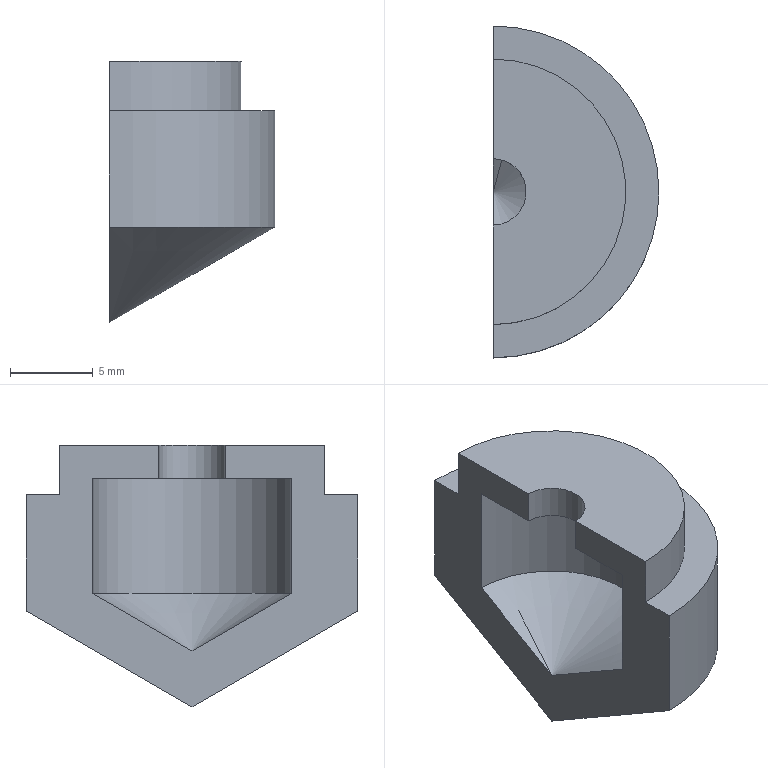Component | NX | VALVE_DISC | 1 solid | 10 faces | box 10 x 20 x 15.77 mm | volume 1233 mm3 | cylinder 4 | plane 4 | cone 2 | commonest cylinder face diameters 20 x1 12 x1 4 x1 16 x1
STEP:
#1=CARTESIAN_POINT('',(0.,0.,0.));
#2=DIRECTION('',(0.,0.,1.));
#3=DIRECTION('',(1.,0.,0.));
#4=AXIS2_PLACEMENT_3D('',#1,#2,#3);
#5=CARTESIAN_POINT('',(-146.777,10.,62.492));
#6=VERTEX_POINT('',#5);
#7=CARTESIAN_POINT('',(-146.777,-10.,62.492));
#8=VERTEX_POINT('',#7);
#9=CARTESIAN_POINT('',(-146.777,0.,62.492));
#10=DIRECTION('',(0.,0.,-1.));
#11=DIRECTION('',(0.,-1.,0.));
#12=AXIS2_PLACEMENT_3D('',#9,#10,#11);
#13=CIRCLE('',#12,10.);
#14=CARTESIAN_POINT('',(-146.777,0.,62.492));
#15=DIRECTION('',(0.,0.,-1.));
#16=DIRECTION('',(0.,-1.,0.));
#17=AXIS2_PLACEMENT_3D('',#14,#15,#16);
#18=CYLINDRICAL_SURFACE('',#17,10.);
#19=CARTESIAN_POINT('',(0.,0.));
#20=DIRECTION('',(1.,0.));
#21=VECTOR('',#20,1.);
#22=LINE('',#19,#21);
#23=(GEOMETRIC_REPRESENTATION_CONTEXT(2)PARAMETRIC_REPRESENTATION_CONTEXT()REPRESENTATION_CONTEXT('',''));
#24=DEFINITIONAL_REPRESENTATION('',(#22),#23);
#25=PCURVE('',#18,#24);
#26=CARTESIAN_POINT('',(-146.777,0.,62.492));
#27=DIRECTION('',(0.,0.,1.));
#28=DIRECTION('',(0.,1.,0.));
#29=AXIS2_PLACEMENT_3D('',#26,#27,#28);
#30=CONICAL_SURFACE('',#29,10.,1.047);
#31=CARTESIAN_POINT('',(9.425,0.));
#32=DIRECTION('',(-1.,0.));
#33=VECTOR('',#32,1.);
#34=LINE('',#31,#33);
#35=(GEOMETRIC_REPRESENTATION_CONTEXT(2)PARAMETRIC_REPRESENTATION_CONTEXT()REPRESENTATION_CONTEXT('',''));
#36=DEFINITIONAL_REPRESENTATION('',(#34),#35);
#37=PCURVE('',#30,#36);
#38=SURFACE_CURVE('',#13,(#25,#37),.PCURVE_S1.);
#39=EDGE_CURVE('',#6,#8,#38,.T.);
#40=ORIENTED_EDGE('',*,*,#39,.F.);
#41=CARTESIAN_POINT('',(-146.777,10.,69.492));
#42=VERTEX_POINT('',#41);
#43=CARTESIAN_POINT('',(-146.777,10.,69.492));
#44=DIRECTION('',(0.,0.,-1.));
#45=VECTOR('',#44,1.);
#46=LINE('',#43,#45);
#47=CARTESIAN_POINT('',(3.142,-7.));
#48=DIRECTION('',(0.,1.));
#49=VECTOR('',#48,1.);
#50=LINE('',#47,#49);
#51=(GEOMETRIC_REPRESENTATION_CONTEXT(2)PARAMETRIC_REPRESENTATION_CONTEXT()REPRESENTATION_CONTEXT('',''));
#52=DEFINITIONAL_REPRESENTATION('',(#50),#51);
#53=PCURVE('',#18,#52);
#54=CARTESIAN_POINT('',(-146.777,0.,62.492));
#55=DIRECTION('',(-1.,0.,0.));
#56=DIRECTION('',(-0.,-1.,0.));
#57=AXIS2_PLACEMENT_3D('',#54,#55,#56);
#58=PLANE('',#57);
#59=CARTESIAN_POINT('',(-10.,7.));
#60=DIRECTION('',(-0.,-1.));
#61=VECTOR('',#60,1.);
#62=LINE('',#59,#61);
#63=(GEOMETRIC_REPRESENTATION_CONTEXT(2)PARAMETRIC_REPRESENTATION_CONTEXT()REPRESENTATION_CONTEXT('',''));
#64=DEFINITIONAL_REPRESENTATION('',(#62),#63);
#65=PCURVE('',#58,#64);
#66=SURFACE_CURVE('',#46,(#53,#65),.PCURVE_S1.);
#67=EDGE_CURVE('',#42,#6,#66,.T.);
#68=ORIENTED_EDGE('',*,*,#67,.F.);
#69=CARTESIAN_POINT('',(-146.777,-10.,69.492));
#70=VERTEX_POINT('',#69);
#71=CARTESIAN_POINT('',(-146.777,0.,69.492));
#72=DIRECTION('',(0.,0.,-1.));
#73=DIRECTION('',(0.,-1.,0.));
#74=AXIS2_PLACEMENT_3D('',#71,#72,#73);
#75=CIRCLE('',#74,10.);
#76=CARTESIAN_POINT('',(0.,-7.));
#77=DIRECTION('',(1.,0.));
#78=VECTOR('',#77,1.);
#79=LINE('',#76,#78);
#80=(GEOMETRIC_REPRESENTATION_CONTEXT(2)PARAMETRIC_REPRESENTATION_CONTEXT()REPRESENTATION_CONTEXT('',''));
#81=DEFINITIONAL_REPRESENTATION('',(#79),#80);
#82=PCURVE('',#18,#81);
#83=CARTESIAN_POINT('',(-146.777,8.,69.492));
#84=DIRECTION('',(0.,0.,-1.));
#85=DIRECTION('',(0.,-1.,0.));
#86=AXIS2_PLACEMENT_3D('',#83,#84,#85);
#87=PLANE('',#86);
#88=CARTESIAN_POINT('',(8.,0.));
#89=DIRECTION('',(1.,0.));
#90=AXIS2_PLACEMENT_2D('',#88,#89);
#91=CIRCLE('',#90,10.);
#92=(GEOMETRIC_REPRESENTATION_CONTEXT(2)PARAMETRIC_REPRESENTATION_CONTEXT()REPRESENTATION_CONTEXT('',''));
#93=DEFINITIONAL_REPRESENTATION('',(#91),#92);
#94=PCURVE('',#87,#93);
#95=SURFACE_CURVE('',#75,(#82,#94),.PCURVE_S1.);
#96=EDGE_CURVE('',#42,#70,#95,.T.);
#97=ORIENTED_EDGE('',*,*,#96,.T.);
#98=CARTESIAN_POINT('',(-146.777,-10.,69.492));
#99=DIRECTION('',(-0.,0.,1.));
#100=VECTOR('',#99,1.);
#101=LINE('',#98,#100);
#102=CARTESIAN_POINT('',(6.283,-7.));
#103=DIRECTION('',(0.,-1.));
#104=VECTOR('',#103,1.);
#105=LINE('',#102,#104);
#106=(GEOMETRIC_REPRESENTATION_CONTEXT(2)PARAMETRIC_REPRESENTATION_CONTEXT()REPRESENTATION_CONTEXT('',''));
#107=DEFINITIONAL_REPRESENTATION('',(#105),#106);
#108=PCURVE('',#18,#107);
#109=CARTESIAN_POINT('',(10.,7.));
#110=DIRECTION('',(-0.,1.));
#111=VECTOR('',#110,1.);
#112=LINE('',#109,#111);
#113=(GEOMETRIC_REPRESENTATION_CONTEXT(2)PARAMETRIC_REPRESENTATION_CONTEXT()REPRESENTATION_CONTEXT('',''));
#114=DEFINITIONAL_REPRESENTATION('',(#112),#113);
#115=PCURVE('',#58,#114);
#116=SURFACE_CURVE('',#101,(#108,#115),.PCURVE_S1.);
#117=EDGE_CURVE('',#8,#70,#116,.T.);
#118=ORIENTED_EDGE('',*,*,#117,.F.);
#119=EDGE_LOOP('',(#40,#68,#97,#118));
#120=FACE_BOUND('',#119,.T.);
#121=ADVANCED_FACE('',(#120),#18,.T.);
#122=CARTESIAN_POINT('',(-146.777,0.,56.718));
#123=VERTEX_POINT('',#122);
#124=CARTESIAN_POINT('',(-146.777,-10.,62.492));
#125=DIRECTION('',(0.,-0.866,0.5));
#126=VECTOR('',#125,1.);
#127=LINE('',#124,#126);
#128=CARTESIAN_POINT('',(3.142,0.));
#129=DIRECTION('',(0.,1.));
#130=VECTOR('',#129,1.);
#131=LINE('',#128,#130);
#132=(GEOMETRIC_REPRESENTATION_CONTEXT(2)PARAMETRIC_REPRESENTATION_CONTEXT()REPRESENTATION_CONTEXT('',''));
#133=DEFINITIONAL_REPRESENTATION('',(#131),#132);
#134=PCURVE('',#30,#133);
#135=CARTESIAN_POINT('',(10.,0.));
#136=DIRECTION('',(0.866,0.5));
#137=VECTOR('',#136,1.);
#138=LINE('',#135,#137);
#139=(GEOMETRIC_REPRESENTATION_CONTEXT(2)PARAMETRIC_REPRESENTATION_CONTEXT()REPRESENTATION_CONTEXT('',''));
#140=DEFINITIONAL_REPRESENTATION('',(#138),#139);
#141=PCURVE('',#58,#140);
#142=SURFACE_CURVE('',#127,(#134,#141),.PCURVE_S1.);
#143=EDGE_CURVE('',#123,#8,#142,.T.);
#144=ORIENTED_EDGE('',*,*,#143,.F.);
#145=CARTESIAN_POINT('',(-146.777,10.,62.492));
#146=DIRECTION('',(-0.,-0.866,-0.5));
#147=VECTOR('',#146,1.);
#148=LINE('',#145,#147);
#149=CARTESIAN_POINT('',(6.283,0.));
#150=DIRECTION('',(0.,-1.));
#151=VECTOR('',#150,1.);
#152=LINE('',#149,#151);
#153=(GEOMETRIC_REPRESENTATION_CONTEXT(2)PARAMETRIC_REPRESENTATION_CONTEXT()REPRESENTATION_CONTEXT('',''));
#154=DEFINITIONAL_REPRESENTATION('',(#152),#153);
#155=PCURVE('',#30,#154);
#156=CARTESIAN_POINT('',(-10.,0.));
#157=DIRECTION('',(0.866,-0.5));
#158=VECTOR('',#157,1.);
#159=LINE('',#156,#158);
#160=(GEOMETRIC_REPRESENTATION_CONTEXT(2)PARAMETRIC_REPRESENTATION_CONTEXT()REPRESENTATION_CONTEXT('',''));
#161=DEFINITIONAL_REPRESENTATION('',(#159),#160);
#162=PCURVE('',#58,#161);
#163=SURFACE_CURVE('',#148,(#155,#162),.PCURVE_S1.);
#164=EDGE_CURVE('',#6,#123,#163,.T.);
#165=ORIENTED_EDGE('',*,*,#164,.F.);
#166=ORIENTED_EDGE('',*,*,#39,.T.);
#167=EDGE_LOOP('',(#144,#165,#166));
#168=FACE_BOUND('',#167,.T.);
#169=ADVANCED_FACE('',(#168),#30,.T.);
#170=CARTESIAN_POINT('',(-146.777,-6.,63.557));
#171=VERTEX_POINT('',#170);
#172=CARTESIAN_POINT('',(-146.777,0.,60.093));
#173=VERTEX_POINT('',#172);
#174=CARTESIAN_POINT('',(-146.777,0.,60.093));
#175=DIRECTION('',(-0.,0.866,-0.5));
#176=VECTOR('',#175,1.);
#177=LINE('',#174,#176);
#178=CARTESIAN_POINT('',(-146.777,0.,60.093));
#179=DIRECTION('',(0.,0.,1.));
#180=DIRECTION('',(0.,1.,0.));
#181=AXIS2_PLACEMENT_3D('',#178,#179,#180);
#182=CONICAL_SURFACE('',#181,0.,1.047);
#183=CARTESIAN_POINT('',(3.142,0.));
#184=DIRECTION('',(0.,-1.));
#185=VECTOR('',#184,1.);
#186=LINE('',#183,#185);
#187=(GEOMETRIC_REPRESENTATION_CONTEXT(2)PARAMETRIC_REPRESENTATION_CONTEXT()REPRESENTATION_CONTEXT('',''));
#188=DEFINITIONAL_REPRESENTATION('',(#186),#187);
#189=PCURVE('',#182,#188);
#190=CARTESIAN_POINT('',(0.,-2.398));
#191=DIRECTION('',(-0.866,-0.5));
#192=VECTOR('',#191,1.);
#193=LINE('',#190,#192);
#194=(GEOMETRIC_REPRESENTATION_CONTEXT(2)PARAMETRIC_REPRESENTATION_CONTEXT()REPRESENTATION_CONTEXT('',''));
#195=DEFINITIONAL_REPRESENTATION('',(#193),#194);
#196=PCURVE('',#58,#195);
#197=SURFACE_CURVE('',#177,(#189,#196),.PCURVE_S1.);
#198=EDGE_CURVE('',#171,#173,#197,.T.);
#199=ORIENTED_EDGE('',*,*,#198,.T.);
#200=CARTESIAN_POINT('',(-146.777,6.,63.557));
#201=VERTEX_POINT('',#200);
#202=CARTESIAN_POINT('',(-146.777,0.,60.093));
#203=DIRECTION('',(0.,0.866,0.5));
#204=VECTOR('',#203,1.);
#205=LINE('',#202,#204);
#206=CARTESIAN_POINT('',(6.283,-0.));
#207=CARTESIAN_POINT('',(6.283,0.05249));
#208=CARTESIAN_POINT('',(6.283,0.1575));
#209=CARTESIAN_POINT('',(6.283,0.3149));
#210=CARTESIAN_POINT('',(6.283,0.4724));
#211=CARTESIAN_POINT('',(6.283,0.6298));
#212=CARTESIAN_POINT('',(6.283,0.7873));
#213=CARTESIAN_POINT('',(6.283,0.9448));
#214=CARTESIAN_POINT('',(6.283,1.102));
#215=CARTESIAN_POINT('',(6.283,1.26));
#216=CARTESIAN_POINT('',(6.283,1.417));
#217=CARTESIAN_POINT('',(6.283,1.575));
#218=CARTESIAN_POINT('',(6.283,1.732));
#219=CARTESIAN_POINT('',(6.283,1.89));
#220=CARTESIAN_POINT('',(6.283,2.047));
#221=CARTESIAN_POINT('',(6.283,2.204));
#222=CARTESIAN_POINT('',(6.283,2.362));
#223=CARTESIAN_POINT('',(6.283,2.519));
#224=CARTESIAN_POINT('',(6.283,2.677));
#225=CARTESIAN_POINT('',(6.283,2.834));
#226=CARTESIAN_POINT('',(6.283,2.992));
#227=CARTESIAN_POINT('',(6.283,3.149));
#228=CARTESIAN_POINT('',(6.283,3.307));
#229=CARTESIAN_POINT('',(6.283,3.412));
#230=CARTESIAN_POINT('',(6.283,3.464));
#231=B_SPLINE_CURVE_WITH_KNOTS('',3,(#206,#207,#208,#209,#210,#211,#212,#213,#214,#215,#216,#217,#218,#219,#220,#221,#222,#223,#224,#225,#226,#227,#228,#229,#230),.UNSPECIFIED.,.F.,.F.,(4,1,1,1,1,1,1,1,1,1,1,1,1,1,1,1,1,1,1,1,1,1,4),(-0.,0.3149,0.6298,0.9448,1.26,1.575,1.89,2.204,2.519,2.834,3.149,3.464,3.779,4.094,4.409,4.724,5.039,5.354,5.669,5.983,6.298,6.613,6.928),.UNSPECIFIED.);
#232=(GEOMETRIC_REPRESENTATION_CONTEXT(2)PARAMETRIC_REPRESENTATION_CONTEXT()REPRESENTATION_CONTEXT('',''));
#233=DEFINITIONAL_REPRESENTATION('',(#231),#232);
#234=PCURVE('',#182,#233);
#235=CARTESIAN_POINT('',(0.,-2.398));
#236=DIRECTION('',(-0.866,0.5));
#237=VECTOR('',#236,1.);
#238=LINE('',#235,#237);
#239=(GEOMETRIC_REPRESENTATION_CONTEXT(2)PARAMETRIC_REPRESENTATION_CONTEXT()REPRESENTATION_CONTEXT('',''));
#240=DEFINITIONAL_REPRESENTATION('',(#238),#239);
#241=PCURVE('',#58,#240);
#242=SURFACE_CURVE('',#205,(#234,#241),.PCURVE_S1.);
#243=EDGE_CURVE('',#173,#201,#242,.T.);
#244=ORIENTED_EDGE('',*,*,#243,.T.);
#245=CARTESIAN_POINT('',(-146.777,0.,63.557));
#246=DIRECTION('',(0.,0.,-1.));
#247=DIRECTION('',(0.,-1.,0.));
#248=AXIS2_PLACEMENT_3D('',#245,#246,#247);
#249=CIRCLE('',#248,6.);
#250=CARTESIAN_POINT('',(9.425,3.464));
#251=DIRECTION('',(-1.,0.));
#252=VECTOR('',#251,1.);
#253=LINE('',#250,#252);
#254=(GEOMETRIC_REPRESENTATION_CONTEXT(2)PARAMETRIC_REPRESENTATION_CONTEXT()REPRESENTATION_CONTEXT('',''));
#255=DEFINITIONAL_REPRESENTATION('',(#253),#254);
#256=PCURVE('',#182,#255);
#257=CARTESIAN_POINT('',(-146.777,0.,62.492));
#258=DIRECTION('',(0.,0.,-1.));
#259=DIRECTION('',(0.,-1.,0.));
#260=AXIS2_PLACEMENT_3D('',#257,#258,#259);
#261=CYLINDRICAL_SURFACE('',#260,6.);
#262=CARTESIAN_POINT('',(0.,-1.066));
#263=DIRECTION('',(1.,0.));
#264=VECTOR('',#263,1.);
#265=LINE('',#262,#264);
#266=(GEOMETRIC_REPRESENTATION_CONTEXT(2)PARAMETRIC_REPRESENTATION_CONTEXT()REPRESENTATION_CONTEXT('',''));
#267=DEFINITIONAL_REPRESENTATION('',(#265),#266);
#268=PCURVE('',#261,#267);
#269=SURFACE_CURVE('',#249,(#256,#268),.PCURVE_S1.);
#270=EDGE_CURVE('',#201,#171,#269,.T.);
#271=ORIENTED_EDGE('',*,*,#270,.T.);
#272=EDGE_LOOP('',(#199,#244,#271));
#273=FACE_BOUND('',#272,.F.);
#274=ADVANCED_FACE('',(#273),#182,.F.);
#275=CARTESIAN_POINT('',(-146.777,-6.,70.492));
#276=VERTEX_POINT('',#275);
#277=CARTESIAN_POINT('',(-146.777,-6.,63.557));
#278=DIRECTION('',(-0.,0.,-1.));
#279=VECTOR('',#278,1.);
#280=LINE('',#277,#279);
#281=CARTESIAN_POINT('',(6.283,-1.066));
#282=DIRECTION('',(0.,1.));
#283=VECTOR('',#282,1.);
#284=LINE('',#281,#283);
#285=(GEOMETRIC_REPRESENTATION_CONTEXT(2)PARAMETRIC_REPRESENTATION_CONTEXT()REPRESENTATION_CONTEXT('',''));
#286=DEFINITIONAL_REPRESENTATION('',(#284),#285);
#287=PCURVE('',#261,#286);
#288=CARTESIAN_POINT('',(6.,1.066));
#289=DIRECTION('',(-0.,-1.));
#290=VECTOR('',#289,1.);
#291=LINE('',#288,#290);
#292=(GEOMETRIC_REPRESENTATION_CONTEXT(2)PARAMETRIC_REPRESENTATION_CONTEXT()REPRESENTATION_CONTEXT('',''));
#293=DEFINITIONAL_REPRESENTATION('',(#291),#292);
#294=PCURVE('',#58,#293);
#295=SURFACE_CURVE('',#280,(#287,#294),.PCURVE_S1.);
#296=EDGE_CURVE('',#276,#171,#295,.T.);
#297=ORIENTED_EDGE('',*,*,#296,.T.);
#298=ORIENTED_EDGE('',*,*,#270,.F.);
#299=CARTESIAN_POINT('',(-146.777,6.,70.492));
#300=VERTEX_POINT('',#299);
#301=CARTESIAN_POINT('',(-146.777,6.,63.557));
#302=DIRECTION('',(0.,0.,1.));
#303=VECTOR('',#302,1.);
#304=LINE('',#301,#303);
#305=CARTESIAN_POINT('',(3.142,-1.066));
#306=DIRECTION('',(0.,-1.));
#307=VECTOR('',#306,1.);
#308=LINE('',#305,#307);
#309=(GEOMETRIC_REPRESENTATION_CONTEXT(2)PARAMETRIC_REPRESENTATION_CONTEXT()REPRESENTATION_CONTEXT('',''));
#310=DEFINITIONAL_REPRESENTATION('',(#308),#309);
#311=PCURVE('',#261,#310);
#312=CARTESIAN_POINT('',(-6.,1.066));
#313=DIRECTION('',(-0.,1.));
#314=VECTOR('',#313,1.);
#315=LINE('',#312,#314);
#316=(GEOMETRIC_REPRESENTATION_CONTEXT(2)PARAMETRIC_REPRESENTATION_CONTEXT()REPRESENTATION_CONTEXT('',''));
#317=DEFINITIONAL_REPRESENTATION('',(#315),#316);
#318=PCURVE('',#58,#317);
#319=SURFACE_CURVE('',#304,(#311,#318),.PCURVE_S1.);
#320=EDGE_CURVE('',#201,#300,#319,.T.);
#321=ORIENTED_EDGE('',*,*,#320,.T.);
#322=CARTESIAN_POINT('',(-146.777,0.,70.492));
#323=DIRECTION('',(0.,0.,-1.));
#324=DIRECTION('',(0.,-1.,0.));
#325=AXIS2_PLACEMENT_3D('',#322,#323,#324);
#326=CIRCLE('',#325,6.);
#327=CARTESIAN_POINT('',(0.,-8.));
#328=DIRECTION('',(1.,0.));
#329=VECTOR('',#328,1.);
#330=LINE('',#327,#329);
#331=(GEOMETRIC_REPRESENTATION_CONTEXT(2)PARAMETRIC_REPRESENTATION_CONTEXT()REPRESENTATION_CONTEXT('',''));
#332=DEFINITIONAL_REPRESENTATION('',(#330),#331);
#333=PCURVE('',#261,#332);
#334=CARTESIAN_POINT('',(-146.777,6.,70.492));
#335=DIRECTION('',(0.,0.,1.));
#336=DIRECTION('',(0.,1.,0.));
#337=AXIS2_PLACEMENT_3D('',#334,#335,#336);
#338=PLANE('',#337);
#339=CARTESIAN_POINT('',(-12.,0.));
#340=CARTESIAN_POINT('',(-12.,10.392));
#341=CARTESIAN_POINT('',(-3.,5.196));
#342=CARTESIAN_POINT('',(6.,0.));
#343=CARTESIAN_POINT('',(-3.,-5.196));
#344=CARTESIAN_POINT('',(-12.,-10.392));
#345=CARTESIAN_POINT('',(-12.,0.));
#346=(BOUNDED_CURVE()B_SPLINE_CURVE(2,(#339,#340,#341,#342,#343,#344,#345),.UNSPECIFIED.,.T.,.F.)B_SPLINE_CURVE_WITH_KNOTS((1,2,2,2,2,1),(-2.094,0.,2.094,4.189,6.283,8.378),.UNSPECIFIED.)CURVE()GEOMETRIC_REPRESENTATION_ITEM()RATIONAL_B_SPLINE_CURVE((1.,0.5,1.,0.5,1.,0.5,1.))REPRESENTATION_ITEM(''));
#347=(GEOMETRIC_REPRESENTATION_CONTEXT(2)PARAMETRIC_REPRESENTATION_CONTEXT()REPRESENTATION_CONTEXT('',''));
#348=DEFINITIONAL_REPRESENTATION('',(#346),#347);
#349=PCURVE('',#338,#348);
#350=SURFACE_CURVE('',#326,(#333,#349),.PCURVE_S1.);
#351=EDGE_CURVE('',#300,#276,#350,.T.);
#352=ORIENTED_EDGE('',*,*,#351,.T.);
#353=EDGE_LOOP('',(#297,#298,#321,#352));
#354=FACE_BOUND('',#353,.F.);
#355=ADVANCED_FACE('',(#354),#261,.F.);
#356=CARTESIAN_POINT('',(-146.777,2.,70.492));
#357=VERTEX_POINT('',#356);
#358=CARTESIAN_POINT('',(-146.777,-2.,70.492));
#359=VERTEX_POINT('',#358);
#360=CARTESIAN_POINT('',(-146.777,0.,70.492));
#361=DIRECTION('',(0.,0.,-1.));
#362=DIRECTION('',(0.,-1.,0.));
#363=AXIS2_PLACEMENT_3D('',#360,#361,#362);
#364=CIRCLE('',#363,2.);
#365=CARTESIAN_POINT('',(-8.,0.));
#366=CARTESIAN_POINT('',(-8.,3.464));
#367=CARTESIAN_POINT('',(-5.,1.732));
#368=CARTESIAN_POINT('',(-2.,0.));
#369=CARTESIAN_POINT('',(-5.,-1.732));
#370=CARTESIAN_POINT('',(-8.,-3.464));
#371=CARTESIAN_POINT('',(-8.,0.));
#372=(BOUNDED_CURVE()B_SPLINE_CURVE(2,(#365,#366,#367,#368,#369,#370,#371),.UNSPECIFIED.,.T.,.F.)B_SPLINE_CURVE_WITH_KNOTS((1,2,2,2,2,1),(-2.094,0.,2.094,4.189,6.283,8.378),.UNSPECIFIED.)CURVE()GEOMETRIC_REPRESENTATION_ITEM()RATIONAL_B_SPLINE_CURVE((1.,0.5,1.,0.5,1.,0.5,1.))REPRESENTATION_ITEM(''));
#373=(GEOMETRIC_REPRESENTATION_CONTEXT(2)PARAMETRIC_REPRESENTATION_CONTEXT()REPRESENTATION_CONTEXT('',''));
#374=DEFINITIONAL_REPRESENTATION('',(#372),#373);
#375=PCURVE('',#338,#374);
#376=CARTESIAN_POINT('',(-146.777,0.,62.492));
#377=DIRECTION('',(0.,0.,-1.));
#378=DIRECTION('',(0.,-1.,0.));
#379=AXIS2_PLACEMENT_3D('',#376,#377,#378);
#380=CYLINDRICAL_SURFACE('',#379,2.);
#381=CARTESIAN_POINT('',(0.,-8.));
#382=DIRECTION('',(1.,0.));
#383=VECTOR('',#382,1.);
#384=LINE('',#381,#383);
#385=(GEOMETRIC_REPRESENTATION_CONTEXT(2)PARAMETRIC_REPRESENTATION_CONTEXT()REPRESENTATION_CONTEXT('',''));
#386=DEFINITIONAL_REPRESENTATION('',(#384),#385);
#387=PCURVE('',#380,#386);
#388=SURFACE_CURVE('',#364,(#375,#387),.PCURVE_S1.);
#389=EDGE_CURVE('',#357,#359,#388,.T.);
#390=ORIENTED_EDGE('',*,*,#389,.F.);
#391=CARTESIAN_POINT('',(-146.777,6.,70.492));
#392=DIRECTION('',(-0.,-1.,-0.));
#393=VECTOR('',#392,1.);
#394=LINE('',#391,#393);
#395=CARTESIAN_POINT('',(0.,0.));
#396=DIRECTION('',(-1.,0.));
#397=VECTOR('',#396,1.);
#398=LINE('',#395,#397);
#399=(GEOMETRIC_REPRESENTATION_CONTEXT(2)PARAMETRIC_REPRESENTATION_CONTEXT()REPRESENTATION_CONTEXT('',''));
#400=DEFINITIONAL_REPRESENTATION('',(#398),#399);
#401=PCURVE('',#338,#400);
#402=CARTESIAN_POINT('',(-6.,8.));
#403=DIRECTION('',(1.,-0.));
#404=VECTOR('',#403,1.);
#405=LINE('',#402,#404);
#406=(GEOMETRIC_REPRESENTATION_CONTEXT(2)PARAMETRIC_REPRESENTATION_CONTEXT()REPRESENTATION_CONTEXT('',''));
#407=DEFINITIONAL_REPRESENTATION('',(#405),#406);
#408=PCURVE('',#58,#407);
#409=SURFACE_CURVE('',#394,(#401,#408),.PCURVE_S1.);
#410=EDGE_CURVE('',#300,#357,#409,.T.);
#411=ORIENTED_EDGE('',*,*,#410,.F.);
#412=ORIENTED_EDGE('',*,*,#351,.T.);
#413=CARTESIAN_POINT('',(-146.777,-6.,70.492));
#414=DIRECTION('',(0.,-1.,0.));
#415=VECTOR('',#414,1.);
#416=LINE('',#413,#415);
#417=CARTESIAN_POINT('',(-12.,0.));
#418=DIRECTION('',(-1.,-0.));
#419=VECTOR('',#418,1.);
#420=LINE('',#417,#419);
#421=(GEOMETRIC_REPRESENTATION_CONTEXT(2)PARAMETRIC_REPRESENTATION_CONTEXT()REPRESENTATION_CONTEXT('',''));
#422=DEFINITIONAL_REPRESENTATION('',(#420),#421);
#423=PCURVE('',#338,#422);
#424=CARTESIAN_POINT('',(6.,8.));
#425=DIRECTION('',(1.,0.));
#426=VECTOR('',#425,1.);
#427=LINE('',#424,#426);
#428=(GEOMETRIC_REPRESENTATION_CONTEXT(2)PARAMETRIC_REPRESENTATION_CONTEXT()REPRESENTATION_CONTEXT('',''));
#429=DEFINITIONAL_REPRESENTATION('',(#427),#428);
#430=PCURVE('',#58,#429);
#431=SURFACE_CURVE('',#416,(#423,#430),.PCURVE_S1.);
#432=EDGE_CURVE('',#359,#276,#431,.T.);
#433=ORIENTED_EDGE('',*,*,#432,.F.);
#434=EDGE_LOOP('',(#390,#411,#412,#433));
#435=FACE_BOUND('',#434,.T.);
#436=ADVANCED_FACE('',(#435),#338,.F.);
#437=CARTESIAN_POINT('',(-146.777,-2.,72.492));
#438=VERTEX_POINT('',#437);
#439=CARTESIAN_POINT('',(-146.777,-2.,70.492));
#440=DIRECTION('',(0.,-0.,-1.));
#441=VECTOR('',#440,1.);
#442=LINE('',#439,#441);
#443=CARTESIAN_POINT('',(6.283,-8.));
#444=DIRECTION('',(0.,1.));
#445=VECTOR('',#444,1.);
#446=LINE('',#443,#445);
#447=(GEOMETRIC_REPRESENTATION_CONTEXT(2)PARAMETRIC_REPRESENTATION_CONTEXT()REPRESENTATION_CONTEXT('',''));
#448=DEFINITIONAL_REPRESENTATION('',(#446),#447);
#449=PCURVE('',#380,#448);
#450=CARTESIAN_POINT('',(2.,8.));
#451=DIRECTION('',(0.,-1.));
#452=VECTOR('',#451,1.);
#453=LINE('',#450,#452);
#454=(GEOMETRIC_REPRESENTATION_CONTEXT(2)PARAMETRIC_REPRESENTATION_CONTEXT()REPRESENTATION_CONTEXT('',''));
#455=DEFINITIONAL_REPRESENTATION('',(#453),#454);
#456=PCURVE('',#58,#455);
#457=SURFACE_CURVE('',#442,(#449,#456),.PCURVE_S1.);
#458=EDGE_CURVE('',#438,#359,#457,.T.);
#459=ORIENTED_EDGE('',*,*,#458,.T.);
#460=ORIENTED_EDGE('',*,*,#389,.F.);
#461=CARTESIAN_POINT('',(-146.777,2.,72.492));
#462=VERTEX_POINT('',#461);
#463=CARTESIAN_POINT('',(-146.777,2.,70.492));
#464=DIRECTION('',(-0.,-0.,1.));
#465=VECTOR('',#464,1.);
#466=LINE('',#463,#465);
#467=CARTESIAN_POINT('',(3.142,-8.));
#468=DIRECTION('',(0.,-1.));
#469=VECTOR('',#468,1.);
#470=LINE('',#467,#469);
#471=(GEOMETRIC_REPRESENTATION_CONTEXT(2)PARAMETRIC_REPRESENTATION_CONTEXT()REPRESENTATION_CONTEXT('',''));
#472=DEFINITIONAL_REPRESENTATION('',(#470),#471);
#473=PCURVE('',#380,#472);
#474=CARTESIAN_POINT('',(-2.,8.));
#475=DIRECTION('',(0.,1.));
#476=VECTOR('',#475,1.);
#477=LINE('',#474,#476);
#478=(GEOMETRIC_REPRESENTATION_CONTEXT(2)PARAMETRIC_REPRESENTATION_CONTEXT()REPRESENTATION_CONTEXT('',''));
#479=DEFINITIONAL_REPRESENTATION('',(#477),#478);
#480=PCURVE('',#58,#479);
#481=SURFACE_CURVE('',#466,(#473,#480),.PCURVE_S1.);
#482=EDGE_CURVE('',#357,#462,#481,.T.);
#483=ORIENTED_EDGE('',*,*,#482,.T.);
#484=CARTESIAN_POINT('',(-146.777,0.,72.492));
#485=DIRECTION('',(0.,0.,-1.));
#486=DIRECTION('',(0.,-1.,0.));
#487=AXIS2_PLACEMENT_3D('',#484,#485,#486);
#488=CIRCLE('',#487,2.);
#489=CARTESIAN_POINT('',(0.,-10.));
#490=DIRECTION('',(1.,0.));
#491=VECTOR('',#490,1.);
#492=LINE('',#489,#491);
#493=(GEOMETRIC_REPRESENTATION_CONTEXT(2)PARAMETRIC_REPRESENTATION_CONTEXT()REPRESENTATION_CONTEXT('',''));
#494=DEFINITIONAL_REPRESENTATION('',(#492),#493);
#495=PCURVE('',#380,#494);
#496=CARTESIAN_POINT('',(-146.777,2.,72.492));
#497=DIRECTION('',(0.,0.,-1.));
#498=DIRECTION('',(0.,-1.,0.));
#499=AXIS2_PLACEMENT_3D('',#496,#497,#498);
#500=PLANE('',#499);
#501=CARTESIAN_POINT('',(2.,0.));
#502=DIRECTION('',(1.,0.));
#503=AXIS2_PLACEMENT_2D('',#501,#502);
#504=CIRCLE('',#503,2.);
#505=(GEOMETRIC_REPRESENTATION_CONTEXT(2)PARAMETRIC_REPRESENTATION_CONTEXT()REPRESENTATION_CONTEXT('',''));
#506=DEFINITIONAL_REPRESENTATION('',(#504),#505);
#507=PCURVE('',#500,#506);
#508=SURFACE_CURVE('',#488,(#495,#507),.PCURVE_S1.);
#509=EDGE_CURVE('',#462,#438,#508,.T.);
#510=ORIENTED_EDGE('',*,*,#509,.T.);
#511=EDGE_LOOP('',(#459,#460,#483,#510));
#512=FACE_BOUND('',#511,.F.);
#513=ADVANCED_FACE('',(#512),#380,.F.);
#514=CARTESIAN_POINT('',(-146.777,8.,72.492));
#515=VERTEX_POINT('',#514);
#516=CARTESIAN_POINT('',(-146.777,-8.,72.492));
#517=VERTEX_POINT('',#516);
#518=CARTESIAN_POINT('',(-146.777,0.,72.492));
#519=DIRECTION('',(0.,0.,-1.));
#520=DIRECTION('',(0.,-1.,0.));
#521=AXIS2_PLACEMENT_3D('',#518,#519,#520);
#522=CIRCLE('',#521,8.);
#523=CARTESIAN_POINT('',(2.,0.));
#524=DIRECTION('',(1.,0.));
#525=AXIS2_PLACEMENT_2D('',#523,#524);
#526=CIRCLE('',#525,8.);
#527=(GEOMETRIC_REPRESENTATION_CONTEXT(2)PARAMETRIC_REPRESENTATION_CONTEXT()REPRESENTATION_CONTEXT('',''));
#528=DEFINITIONAL_REPRESENTATION('',(#526),#527);
#529=PCURVE('',#500,#528);
#530=CARTESIAN_POINT('',(-146.777,0.,62.492));
#531=DIRECTION('',(0.,0.,-1.));
#532=DIRECTION('',(0.,-1.,0.));
#533=AXIS2_PLACEMENT_3D('',#530,#531,#532);
#534=CYLINDRICAL_SURFACE('',#533,8.);
#535=CARTESIAN_POINT('',(0.,-10.));
#536=DIRECTION('',(1.,0.));
#537=VECTOR('',#536,1.);
#538=LINE('',#535,#537);
#539=(GEOMETRIC_REPRESENTATION_CONTEXT(2)PARAMETRIC_REPRESENTATION_CONTEXT()REPRESENTATION_CONTEXT('',''));
#540=DEFINITIONAL_REPRESENTATION('',(#538),#539);
#541=PCURVE('',#534,#540);
#542=SURFACE_CURVE('',#522,(#529,#541),.PCURVE_S1.);
#543=EDGE_CURVE('',#515,#517,#542,.T.);
#544=ORIENTED_EDGE('',*,*,#543,.F.);
#545=CARTESIAN_POINT('',(-146.777,2.,72.492));
#546=DIRECTION('',(0.,1.,0.));
#547=VECTOR('',#546,1.);
#548=LINE('',#545,#547);
#549=CARTESIAN_POINT('',(0.,0.));
#550=DIRECTION('',(-1.,-0.));
#551=VECTOR('',#550,1.);
#552=LINE('',#549,#551);
#553=(GEOMETRIC_REPRESENTATION_CONTEXT(2)PARAMETRIC_REPRESENTATION_CONTEXT()REPRESENTATION_CONTEXT('',''));
#554=DEFINITIONAL_REPRESENTATION('',(#552),#553);
#555=PCURVE('',#500,#554);
#556=CARTESIAN_POINT('',(-2.,10.));
#557=DIRECTION('',(-1.,0.));
#558=VECTOR('',#557,1.);
#559=LINE('',#556,#558);
#560=(GEOMETRIC_REPRESENTATION_CONTEXT(2)PARAMETRIC_REPRESENTATION_CONTEXT()REPRESENTATION_CONTEXT('',''));
#561=DEFINITIONAL_REPRESENTATION('',(#559),#560);
#562=PCURVE('',#58,#561);
#563=SURFACE_CURVE('',#548,(#555,#562),.PCURVE_S1.);
#564=EDGE_CURVE('',#462,#515,#563,.T.);
#565=ORIENTED_EDGE('',*,*,#564,.F.);
#566=ORIENTED_EDGE('',*,*,#509,.T.);
#567=CARTESIAN_POINT('',(-146.777,-2.,72.492));
#568=DIRECTION('',(-0.,1.,-0.));
#569=VECTOR('',#568,1.);
#570=LINE('',#567,#569);
#571=CARTESIAN_POINT('',(4.,0.));
#572=DIRECTION('',(-1.,0.));
#573=VECTOR('',#572,1.);
#574=LINE('',#571,#573);
#575=(GEOMETRIC_REPRESENTATION_CONTEXT(2)PARAMETRIC_REPRESENTATION_CONTEXT()REPRESENTATION_CONTEXT('',''));
#576=DEFINITIONAL_REPRESENTATION('',(#574),#575);
#577=PCURVE('',#500,#576);
#578=CARTESIAN_POINT('',(2.,10.));
#579=DIRECTION('',(-1.,-0.));
#580=VECTOR('',#579,1.);
#581=LINE('',#578,#580);
#582=(GEOMETRIC_REPRESENTATION_CONTEXT(2)PARAMETRIC_REPRESENTATION_CONTEXT()REPRESENTATION_CONTEXT('',''));
#583=DEFINITIONAL_REPRESENTATION('',(#581),#582);
#584=PCURVE('',#58,#583);
#585=SURFACE_CURVE('',#570,(#577,#584),.PCURVE_S1.);
#586=EDGE_CURVE('',#517,#438,#585,.T.);
#587=ORIENTED_EDGE('',*,*,#586,.F.);
#588=EDGE_LOOP('',(#544,#565,#566,#587));
#589=FACE_BOUND('',#588,.T.);
#590=ADVANCED_FACE('',(#589),#500,.F.);
#591=CARTESIAN_POINT('',(-146.777,8.,69.492));
#592=VERTEX_POINT('',#591);
#593=CARTESIAN_POINT('',(-146.777,-8.,69.492));
#594=VERTEX_POINT('',#593);
#595=CARTESIAN_POINT('',(-146.777,0.,69.492));
#596=DIRECTION('',(0.,0.,-1.));
#597=DIRECTION('',(0.,-1.,0.));
#598=AXIS2_PLACEMENT_3D('',#595,#596,#597);
#599=CIRCLE('',#598,8.);
#600=CARTESIAN_POINT('',(0.,-7.));
#601=DIRECTION('',(1.,0.));
#602=VECTOR('',#601,1.);
#603=LINE('',#600,#602);
#604=(GEOMETRIC_REPRESENTATION_CONTEXT(2)PARAMETRIC_REPRESENTATION_CONTEXT()REPRESENTATION_CONTEXT('',''));
#605=DEFINITIONAL_REPRESENTATION('',(#603),#604);
#606=PCURVE('',#534,#605);
#607=CARTESIAN_POINT('',(8.,0.));
#608=DIRECTION('',(1.,0.));
#609=AXIS2_PLACEMENT_2D('',#607,#608);
#610=CIRCLE('',#609,8.);
#611=(GEOMETRIC_REPRESENTATION_CONTEXT(2)PARAMETRIC_REPRESENTATION_CONTEXT()REPRESENTATION_CONTEXT('',''));
#612=DEFINITIONAL_REPRESENTATION('',(#610),#611);
#613=PCURVE('',#87,#612);
#614=SURFACE_CURVE('',#599,(#606,#613),.PCURVE_S1.);
#615=EDGE_CURVE('',#592,#594,#614,.T.);
#616=ORIENTED_EDGE('',*,*,#615,.F.);
#617=CARTESIAN_POINT('',(-146.777,8.,72.492));
#618=DIRECTION('',(0.,0.,-1.));
#619=VECTOR('',#618,1.);
#620=LINE('',#617,#619);
#621=CARTESIAN_POINT('',(3.142,-10.));
#622=DIRECTION('',(0.,1.));
#623=VECTOR('',#622,1.);
#624=LINE('',#621,#623);
#625=(GEOMETRIC_REPRESENTATION_CONTEXT(2)PARAMETRIC_REPRESENTATION_CONTEXT()REPRESENTATION_CONTEXT('',''));
#626=DEFINITIONAL_REPRESENTATION('',(#624),#625);
#627=PCURVE('',#534,#626);
#628=CARTESIAN_POINT('',(-8.,10.));
#629=DIRECTION('',(-0.,-1.));
#630=VECTOR('',#629,1.);
#631=LINE('',#628,#630);
#632=(GEOMETRIC_REPRESENTATION_CONTEXT(2)PARAMETRIC_REPRESENTATION_CONTEXT()REPRESENTATION_CONTEXT('',''));
#633=DEFINITIONAL_REPRESENTATION('',(#631),#632);
#634=PCURVE('',#58,#633);
#635=SURFACE_CURVE('',#620,(#627,#634),.PCURVE_S1.);
#636=EDGE_CURVE('',#515,#592,#635,.T.);
#637=ORIENTED_EDGE('',*,*,#636,.F.);
#638=ORIENTED_EDGE('',*,*,#543,.T.);
#639=CARTESIAN_POINT('',(-146.777,-8.,72.492));
#640=DIRECTION('',(-0.,0.,1.));
#641=VECTOR('',#640,1.);
#642=LINE('',#639,#641);
#643=CARTESIAN_POINT('',(6.283,-10.));
#644=DIRECTION('',(0.,-1.));
#645=VECTOR('',#644,1.);
#646=LINE('',#643,#645);
#647=(GEOMETRIC_REPRESENTATION_CONTEXT(2)PARAMETRIC_REPRESENTATION_CONTEXT()REPRESENTATION_CONTEXT('',''));
#648=DEFINITIONAL_REPRESENTATION('',(#646),#647);
#649=PCURVE('',#534,#648);
#650=CARTESIAN_POINT('',(8.,10.));
#651=DIRECTION('',(-0.,1.));
#652=VECTOR('',#651,1.);
#653=LINE('',#650,#652);
#654=(GEOMETRIC_REPRESENTATION_CONTEXT(2)PARAMETRIC_REPRESENTATION_CONTEXT()REPRESENTATION_CONTEXT('',''));
#655=DEFINITIONAL_REPRESENTATION('',(#653),#654);
#656=PCURVE('',#58,#655);
#657=SURFACE_CURVE('',#642,(#649,#656),.PCURVE_S1.);
#658=EDGE_CURVE('',#594,#517,#657,.T.);
#659=ORIENTED_EDGE('',*,*,#658,.F.);
#660=EDGE_LOOP('',(#616,#637,#638,#659));
#661=FACE_BOUND('',#660,.T.);
#662=ADVANCED_FACE('',(#661),#534,.T.);
#663=CARTESIAN_POINT('',(-146.777,8.,69.492));
#664=DIRECTION('',(0.,1.,0.));
#665=VECTOR('',#664,1.);
#666=LINE('',#663,#665);
#667=CARTESIAN_POINT('',(0.,0.));
#668=DIRECTION('',(-1.,-0.));
#669=VECTOR('',#668,1.);
#670=LINE('',#667,#669);
#671=(GEOMETRIC_REPRESENTATION_CONTEXT(2)PARAMETRIC_REPRESENTATION_CONTEXT()REPRESENTATION_CONTEXT('',''));
#672=DEFINITIONAL_REPRESENTATION('',(#670),#671);
#673=PCURVE('',#87,#672);
#674=CARTESIAN_POINT('',(-8.,7.));
#675=DIRECTION('',(-1.,0.));
#676=VECTOR('',#675,1.);
#677=LINE('',#674,#676);
#678=(GEOMETRIC_REPRESENTATION_CONTEXT(2)PARAMETRIC_REPRESENTATION_CONTEXT()REPRESENTATION_CONTEXT('',''));
#679=DEFINITIONAL_REPRESENTATION('',(#677),#678);
#680=PCURVE('',#58,#679);
#681=SURFACE_CURVE('',#666,(#673,#680),.PCURVE_S1.);
#682=EDGE_CURVE('',#592,#42,#681,.T.);
#683=ORIENTED_EDGE('',*,*,#682,.F.);
#684=ORIENTED_EDGE('',*,*,#615,.T.);
#685=CARTESIAN_POINT('',(-146.777,-8.,69.492));
#686=DIRECTION('',(-0.,1.,-0.));
#687=VECTOR('',#686,1.);
#688=LINE('',#685,#687);
#689=CARTESIAN_POINT('',(16.,0.));
#690=DIRECTION('',(-1.,0.));
#691=VECTOR('',#690,1.);
#692=LINE('',#689,#691);
#693=(GEOMETRIC_REPRESENTATION_CONTEXT(2)PARAMETRIC_REPRESENTATION_CONTEXT()REPRESENTATION_CONTEXT('',''));
#694=DEFINITIONAL_REPRESENTATION('',(#692),#693);
#695=PCURVE('',#87,#694);
#696=CARTESIAN_POINT('',(8.,7.));
#697=DIRECTION('',(-1.,-0.));
#698=VECTOR('',#697,1.);
#699=LINE('',#696,#698);
#700=(GEOMETRIC_REPRESENTATION_CONTEXT(2)PARAMETRIC_REPRESENTATION_CONTEXT()REPRESENTATION_CONTEXT('',''));
#701=DEFINITIONAL_REPRESENTATION('',(#699),#700);
#702=PCURVE('',#58,#701);
#703=SURFACE_CURVE('',#688,(#695,#702),.PCURVE_S1.);
#704=EDGE_CURVE('',#70,#594,#703,.T.);
#705=ORIENTED_EDGE('',*,*,#704,.F.);
#706=ORIENTED_EDGE('',*,*,#96,.F.);
#707=EDGE_LOOP('',(#683,#684,#705,#706));
#708=FACE_BOUND('',#707,.T.);
#709=ADVANCED_FACE('',(#708),#87,.F.);
#710=ORIENTED_EDGE('',*,*,#67,.T.);
#711=ORIENTED_EDGE('',*,*,#164,.T.);
#712=ORIENTED_EDGE('',*,*,#143,.T.);
#713=ORIENTED_EDGE('',*,*,#117,.T.);
#714=ORIENTED_EDGE('',*,*,#704,.T.);
#715=ORIENTED_EDGE('',*,*,#658,.T.);
#716=ORIENTED_EDGE('',*,*,#586,.T.);
#717=ORIENTED_EDGE('',*,*,#458,.T.);
#718=ORIENTED_EDGE('',*,*,#432,.T.);
#719=ORIENTED_EDGE('',*,*,#296,.T.);
#720=ORIENTED_EDGE('',*,*,#198,.T.);
#721=ORIENTED_EDGE('',*,*,#243,.T.);
#722=ORIENTED_EDGE('',*,*,#320,.T.);
#723=ORIENTED_EDGE('',*,*,#410,.T.);
#724=ORIENTED_EDGE('',*,*,#482,.T.);
#725=ORIENTED_EDGE('',*,*,#564,.T.);
#726=ORIENTED_EDGE('',*,*,#636,.T.);
#727=ORIENTED_EDGE('',*,*,#682,.T.);
#728=EDGE_LOOP('',(#710,#711,#712,#713,#714,#715,#716,#717,#718,#719,#720,#721,#722,#723,#724,#725,#726,#727));
#729=FACE_BOUND('',#728,.T.);
#730=ADVANCED_FACE('',(#729),#58,.T.);
#731=CLOSED_SHELL('',(#121,#169,#274,#355,#436,#513,#590,#662,#709,#730));
#732=MANIFOLD_SOLID_BREP('',#731);
#733=(LENGTH_UNIT()NAMED_UNIT(*)SI_UNIT(.MILLI.,.METRE.));
#734=UNCERTAINTY_MEASURE_WITH_UNIT(LENGTH_MEASURE(0.0000001),#733,'','');
#735=(NAMED_UNIT(*)PLANE_ANGLE_UNIT()SI_UNIT($,.RADIAN.));
#736=(NAMED_UNIT(*)SI_UNIT($,.STERADIAN.)SOLID_ANGLE_UNIT());
#737=(GEOMETRIC_REPRESENTATION_CONTEXT(3)GLOBAL_UNCERTAINTY_ASSIGNED_CONTEXT((#734))GLOBAL_UNIT_ASSIGNED_CONTEXT((#733,#735,#736))REPRESENTATION_CONTEXT('',''));
#738=ADVANCED_BREP_SHAPE_REPRESENTATION('',(#4,#732),#737);